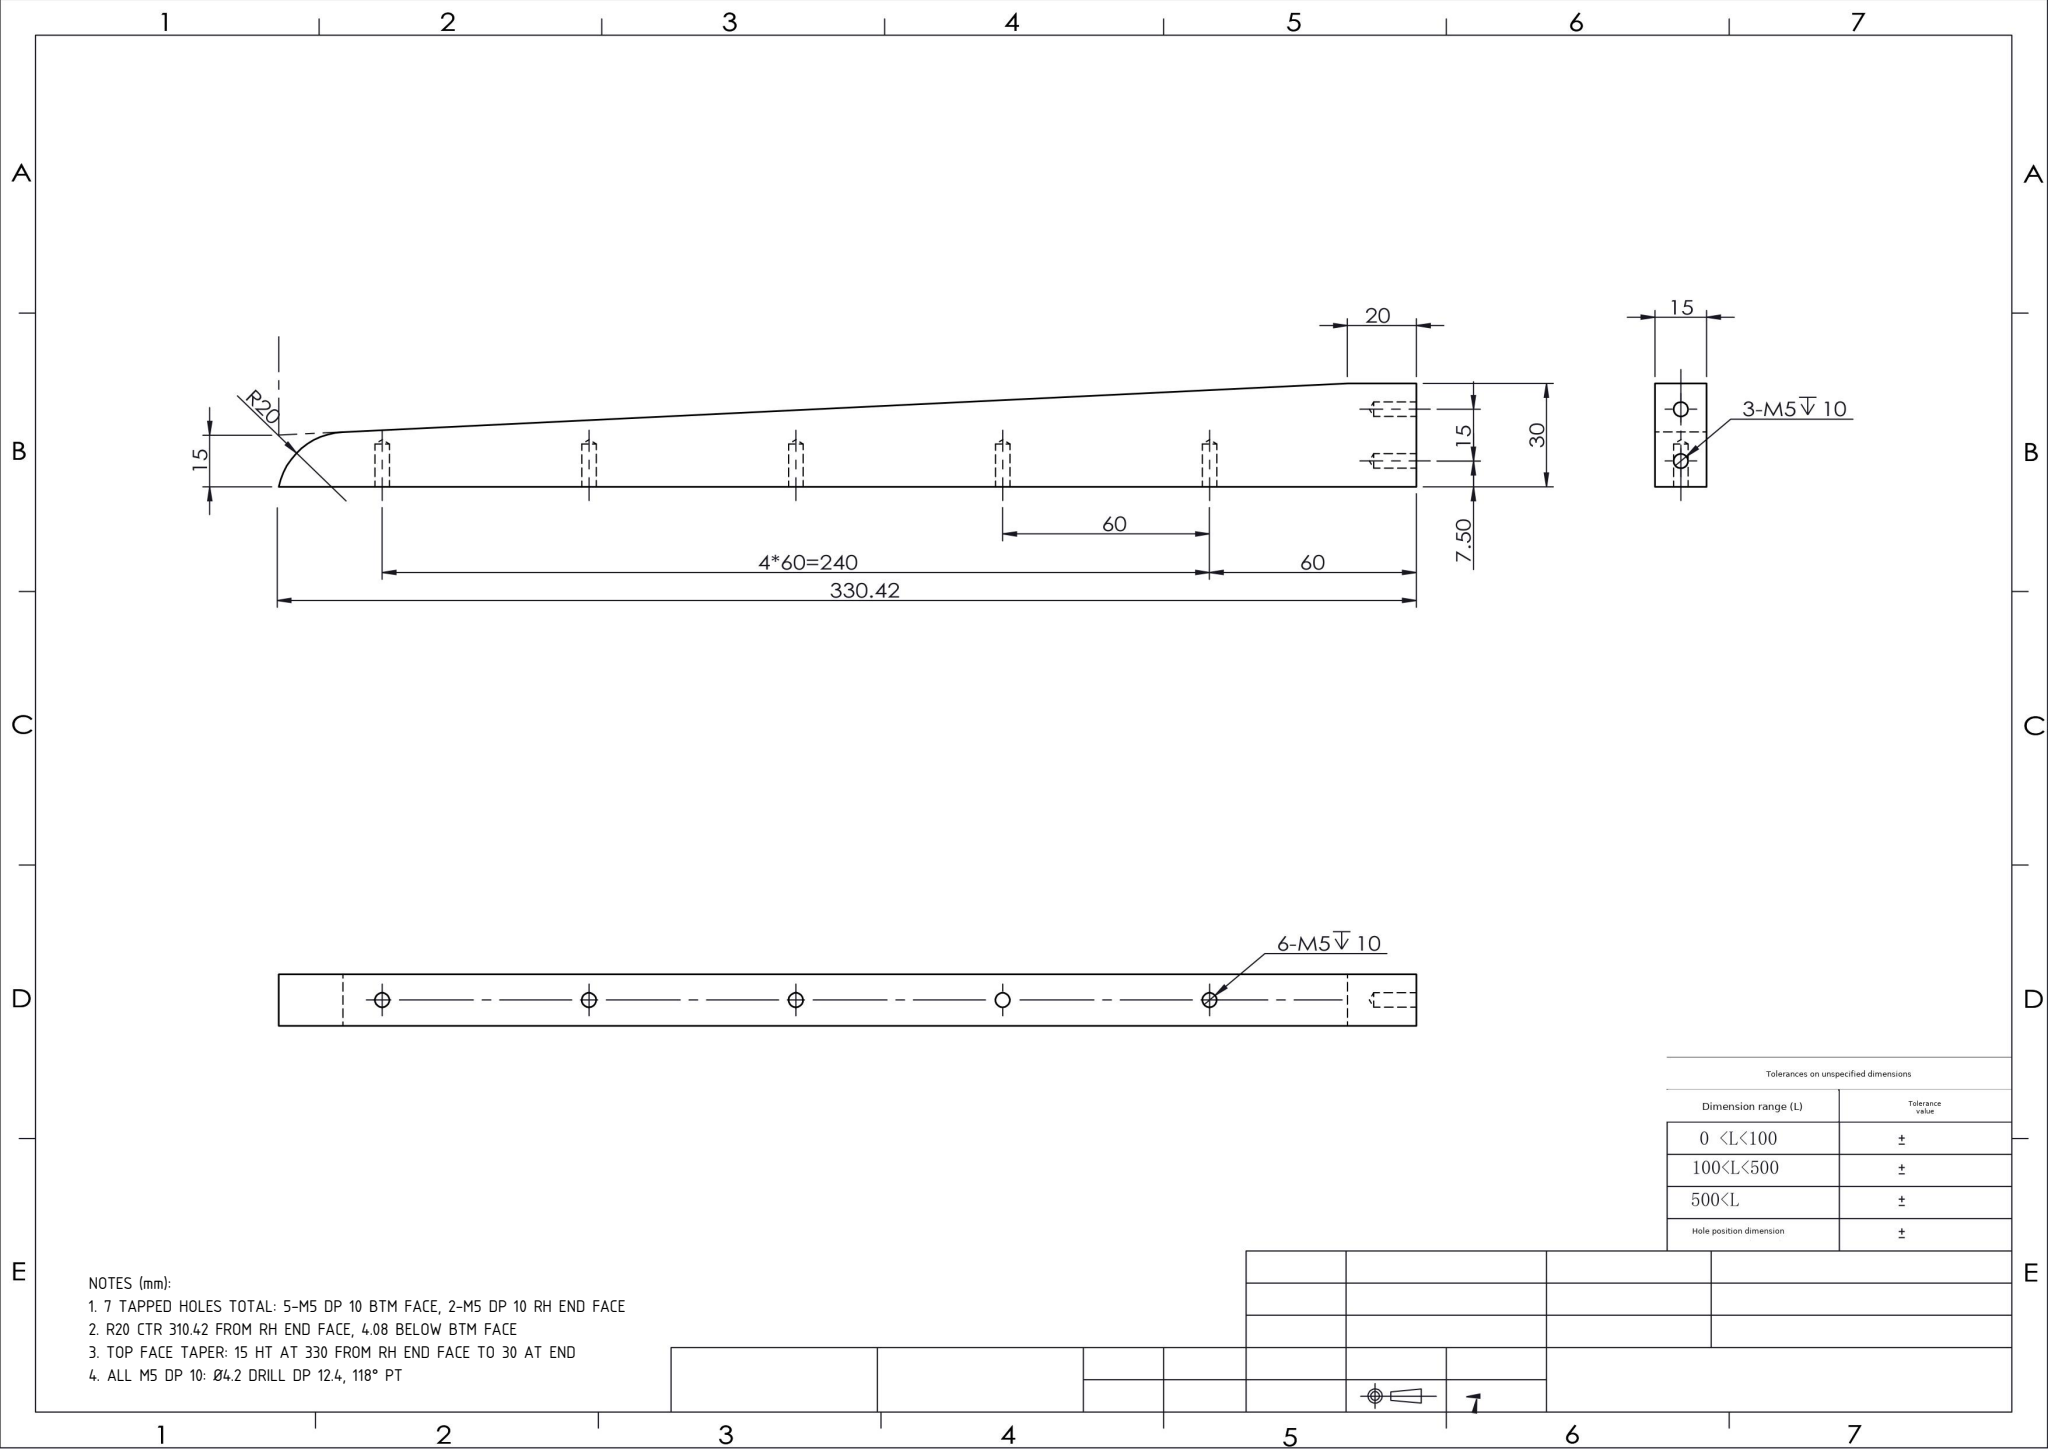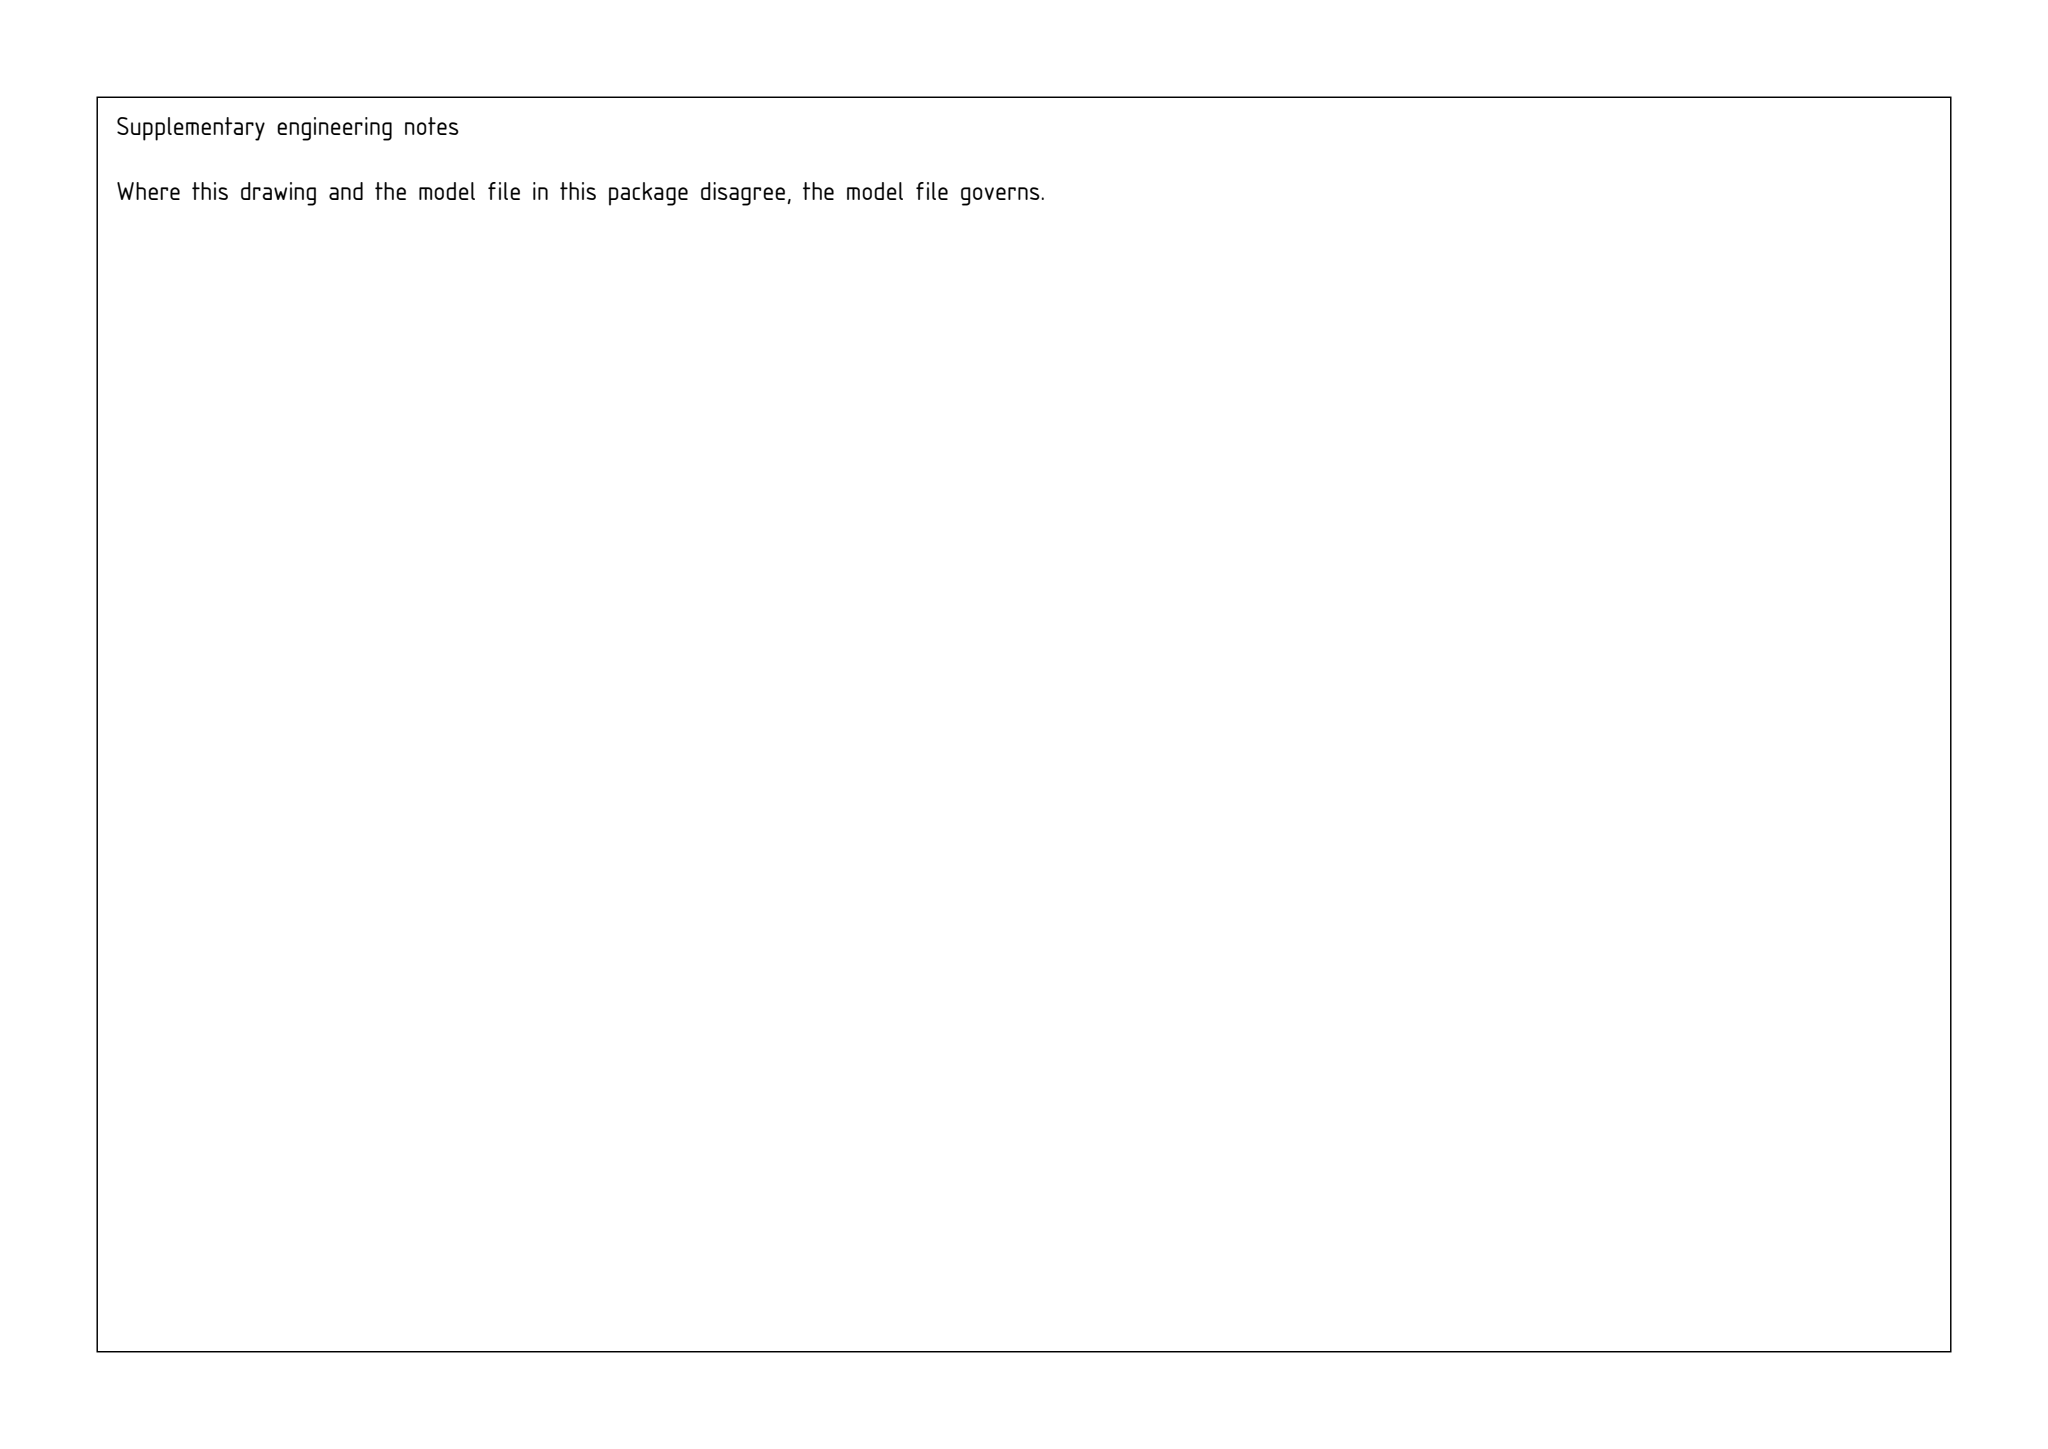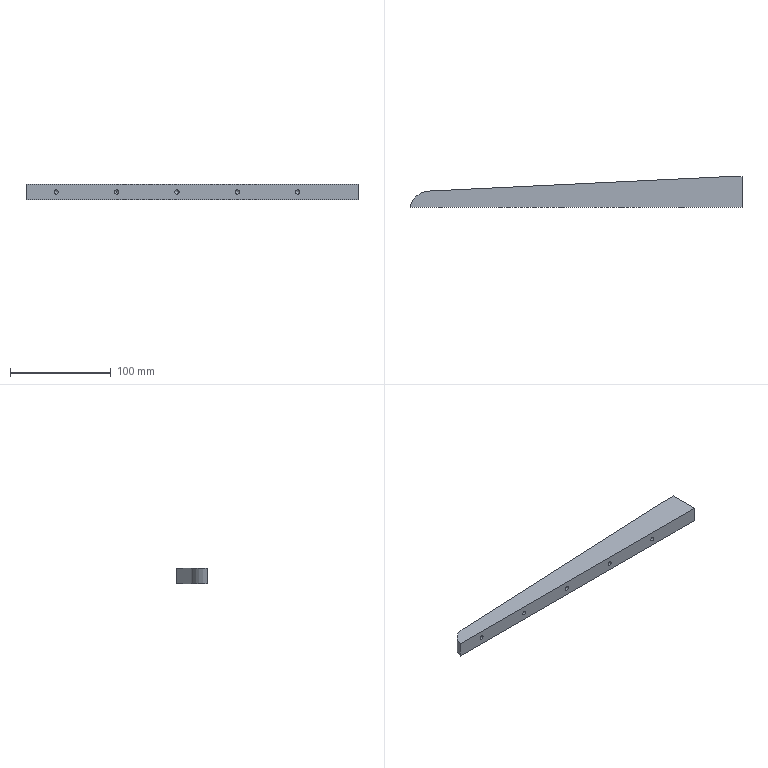Part | SolidWorks | mm | 1 solid | 35 faces | box 330 x 30 x 15 mm | volume 111335 mm3 | cylinder 15 | cone 14 | plane 6 | commonest cylinder face diameters 4.2 x14 40 x1
Drawing notes:
7 TAPPED HOLES TOTAL: 5-M5 DP 10 BTM FACE, 2-M5 DP 10 RH END FACE | from the solid: Y-axis Ø4.2 holes at x=30,90,150,210,270 (z=7.5) = 5; X-axis Ø4.2 holes at y=7.5 & 22.5 (z=7.5) = 2
R20 CTR 310.42 FROM RH END FACE, 4.08 BELOW BTM FACE | from the solid: Ø40 cyl, axis z, ctr (19.58,-4.08); RH end face plane x=330 -> 330-19.58=310.42; btm face y=0
TOP FACE TAPER: 15 HT AT 330 FROM RH END FACE TO 30 AT END | from the solid: bbox 330x30x15; sloped face tangent to R20 at ctr(19.58,-4.08); ht 15 at x=0, 30 at x=330
ALL M5 DP 10: Ø4.2 DRILL DP 12.4, 118° PT | from the solid: cylinders dia 4.2 length 12.4; cones included angle 118.0 ref dia 4.2